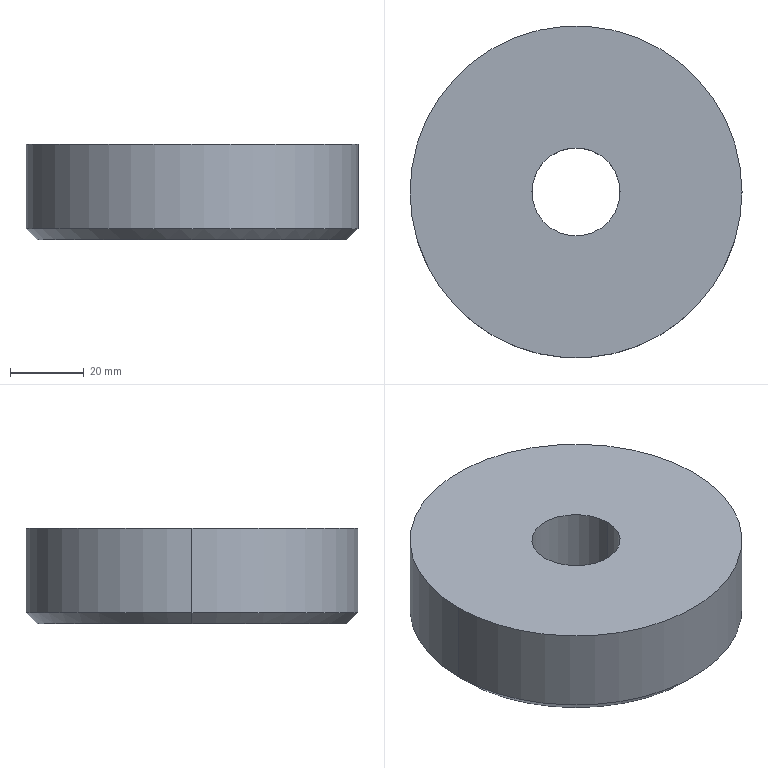Component | SolidWorks | PolishingHead-1 | 1 solid | 8 faces | box 90.34 x 90.34 x 26 mm | volume 153646 mm3 | cylinder 4 | cone 2 | plane 2 | commonest cylinder face diameters 24 x2 90.34 x2
build123d program:
from build123d import *

# Parameters (mm, degrees)
SKETCH1_R           = 45.17
BOSS_EXTRUDE1_DEPTH = 26
CHAMFER1_SIZE       = 3
SKETCH2_R           = 12
CUT_EXTRUDE1_DEPTH  = 26


with BuildPart() as part:
    # Sketch1 → Boss-Extrude1 (new body)
    with BuildSketch(Plane.XY):
        Circle(SKETCH1_R)
    extrude(amount=BOSS_EXTRUDE1_DEPTH)

    # Chamfer1
    chamfer1_edges = [part.edges().sort_by_distance(p)[0] for p in [
        (-45.17, 0, 26),
    ]]
    chamfer(chamfer1_edges, length=CHAMFER1_SIZE)

    # Sketch2 → Cut-Extrude1 (cut)
    with BuildSketch(Plane.XY.offset(26)):
        Circle(SKETCH2_R)
    extrude(amount=-CUT_EXTRUDE1_DEPTH, mode=Mode.SUBTRACT)


solid = part.part

# Placed as in the assembly
solid = solid.moved(Location((0, 0, -90), (180, 0, 0)))
STEP:
#1=CARTESIAN_POINT('',(0.4724,0.,-3.543));
#2=VERTEX_POINT('',#1);
#3=CARTESIAN_POINT('',(-0.4724,0.,-3.543));
#4=VERTEX_POINT('',#3);
#5=CARTESIAN_POINT('',(0.,0.,-3.543));
#6=DIRECTION('',(0.,0.,-1.));
#7=DIRECTION('',(-1.,0.,0.));
#8=AXIS2_PLACEMENT_3D('',#5,#6,#7);
#9=CIRCLE('',#8,0.4724);
#10=EDGE_CURVE('',#2,#4,#9,.T.);
#11=ORIENTED_EDGE('',*,*,#10,.F.);
#12=CARTESIAN_POINT('',(0.4724,0.,-4.567));
#13=VERTEX_POINT('',#12);
#14=CARTESIAN_POINT('',(0.4724,0.,-3.543));
#15=DIRECTION('',(0.,0.,-1.));
#16=VECTOR('',#15,39.37);
#17=LINE('',#14,#16);
#18=EDGE_CURVE('',#2,#13,#17,.T.);
#19=ORIENTED_EDGE('',*,*,#18,.T.);
#20=CARTESIAN_POINT('',(-0.4724,0.,-4.567));
#21=VERTEX_POINT('',#20);
#22=CARTESIAN_POINT('',(0.,0.,-4.567));
#23=DIRECTION('',(0.,0.,-1.));
#24=DIRECTION('',(-1.,0.,0.));
#25=AXIS2_PLACEMENT_3D('',#22,#23,#24);
#26=CIRCLE('',#25,0.4724);
#27=EDGE_CURVE('',#13,#21,#26,.T.);
#28=ORIENTED_EDGE('',*,*,#27,.T.);
#29=CARTESIAN_POINT('',(-0.4724,0.,-3.543));
#30=DIRECTION('',(0.,0.,-1.));
#31=VECTOR('',#30,39.37);
#32=LINE('',#29,#31);
#33=EDGE_CURVE('',#4,#21,#32,.T.);
#34=ORIENTED_EDGE('',*,*,#33,.F.);
#35=EDGE_LOOP('',(#11,#19,#28,#34));
#36=FACE_OUTER_BOUND('',#35,.T.);
#37=CARTESIAN_POINT('',(0.,0.,-3.543));
#38=DIRECTION('',(0.,0.,-1.));
#39=DIRECTION('',(-1.,0.,0.));
#40=AXIS2_PLACEMENT_3D('',#37,#38,#39);
#41=CYLINDRICAL_SURFACE('',#40,0.4724);
#42=ADVANCED_FACE('',(#36),#41,.F.);
#43=CARTESIAN_POINT('',(-1.66,0.,-4.567));
#44=VERTEX_POINT('',#43);
#45=CARTESIAN_POINT('',(1.66,0.,-4.567));
#46=VERTEX_POINT('',#45);
#47=CARTESIAN_POINT('',(0.,0.,-4.567));
#48=DIRECTION('',(0.,0.,-1.));
#49=DIRECTION('',(-1.,0.,0.));
#50=AXIS2_PLACEMENT_3D('',#47,#48,#49);
#51=CIRCLE('',#50,1.66);
#52=EDGE_CURVE('',#44,#46,#51,.T.);
#53=ORIENTED_EDGE('',*,*,#52,.F.);
#54=CARTESIAN_POINT('',(-1.778,0.,-4.449));
#55=VERTEX_POINT('',#54);
#56=CARTESIAN_POINT('',(-1.66,0.,-4.567));
#57=DIRECTION('',(-0.7071,0.,0.7071));
#58=VECTOR('',#57,39.37);
#59=LINE('',#56,#58);
#60=EDGE_CURVE('',#44,#55,#59,.T.);
#61=ORIENTED_EDGE('',*,*,#60,.T.);
#62=CARTESIAN_POINT('',(1.778,0.,-4.449));
#63=VERTEX_POINT('',#62);
#64=CARTESIAN_POINT('',(0.,0.,-4.449));
#65=DIRECTION('',(0.,0.,1.));
#66=DIRECTION('',(-1.,0.,0.));
#67=AXIS2_PLACEMENT_3D('',#64,#65,#66);
#68=CIRCLE('',#67,1.778);
#69=EDGE_CURVE('',#63,#55,#68,.T.);
#70=ORIENTED_EDGE('',*,*,#69,.F.);
#71=CARTESIAN_POINT('',(1.66,0.,-4.567));
#72=DIRECTION('',(0.7071,0.,0.7071));
#73=VECTOR('',#72,39.37);
#74=LINE('',#71,#73);
#75=EDGE_CURVE('',#46,#63,#74,.T.);
#76=ORIENTED_EDGE('',*,*,#75,.F.);
#77=EDGE_LOOP('',(#53,#61,#70,#76));
#78=FACE_OUTER_BOUND('',#77,.T.);
#79=CARTESIAN_POINT('',(0.,0.,-4.567));
#80=DIRECTION('',(0.,0.,1.));
#81=DIRECTION('',(1.,0.,0.));
#82=AXIS2_PLACEMENT_3D('',#79,#80,#81);
#83=CONICAL_SURFACE('',#82,1.66,0.7854);
#84=ADVANCED_FACE('',(#78),#83,.T.);
#85=ORIENTED_EDGE('',*,*,#69,.T.);
#86=CARTESIAN_POINT('',(-1.778,0.,-3.543));
#87=VERTEX_POINT('',#86);
#88=CARTESIAN_POINT('',(-1.778,0.,-4.567));
#89=DIRECTION('',(0.,0.,1.));
#90=VECTOR('',#89,39.37);
#91=LINE('',#88,#90);
#92=EDGE_CURVE('',#55,#87,#91,.T.);
#93=ORIENTED_EDGE('',*,*,#92,.T.);
#94=CARTESIAN_POINT('',(1.778,0.,-3.543));
#95=VERTEX_POINT('',#94);
#96=CARTESIAN_POINT('',(0.,0.,-3.543));
#97=DIRECTION('',(0.,0.,-1.));
#98=DIRECTION('',(-1.,0.,0.));
#99=AXIS2_PLACEMENT_3D('',#96,#97,#98);
#100=CIRCLE('',#99,1.778);
#101=EDGE_CURVE('',#87,#95,#100,.T.);
#102=ORIENTED_EDGE('',*,*,#101,.T.);
#103=CARTESIAN_POINT('',(1.778,0.,-4.567));
#104=DIRECTION('',(0.,0.,1.));
#105=VECTOR('',#104,39.37);
#106=LINE('',#103,#105);
#107=EDGE_CURVE('',#63,#95,#106,.T.);
#108=ORIENTED_EDGE('',*,*,#107,.F.);
#109=EDGE_LOOP('',(#85,#93,#102,#108));
#110=FACE_OUTER_BOUND('',#109,.T.);
#111=CARTESIAN_POINT('',(0.,0.,-4.567));
#112=DIRECTION('',(0.,0.,1.));
#113=DIRECTION('',(1.,0.,0.));
#114=AXIS2_PLACEMENT_3D('',#111,#112,#113);
#115=CYLINDRICAL_SURFACE('',#114,1.778);
#116=ADVANCED_FACE('',(#110),#115,.T.);
#117=ORIENTED_EDGE('',*,*,#92,.F.);
#118=CARTESIAN_POINT('',(0.,0.,-4.449));
#119=DIRECTION('',(0.,0.,1.));
#120=DIRECTION('',(-1.,0.,0.));
#121=AXIS2_PLACEMENT_3D('',#118,#119,#120);
#122=CIRCLE('',#121,1.778);
#123=EDGE_CURVE('',#55,#63,#122,.T.);
#124=ORIENTED_EDGE('',*,*,#123,.T.);
#125=ORIENTED_EDGE('',*,*,#107,.T.);
#126=CARTESIAN_POINT('',(0.,0.,-3.543));
#127=DIRECTION('',(0.,0.,-1.));
#128=DIRECTION('',(-1.,0.,0.));
#129=AXIS2_PLACEMENT_3D('',#126,#127,#128);
#130=CIRCLE('',#129,1.778);
#131=EDGE_CURVE('',#95,#87,#130,.T.);
#132=ORIENTED_EDGE('',*,*,#131,.T.);
#133=EDGE_LOOP('',(#117,#124,#125,#132));
#134=FACE_OUTER_BOUND('',#133,.T.);
#135=CARTESIAN_POINT('',(0.,0.,-4.567));
#136=DIRECTION('',(0.,0.,1.));
#137=DIRECTION('',(1.,0.,0.));
#138=AXIS2_PLACEMENT_3D('',#135,#136,#137);
#139=CYLINDRICAL_SURFACE('',#138,1.778);
#140=ADVANCED_FACE('',(#134),#139,.T.);
#141=CARTESIAN_POINT('',(0.,0.,-4.567));
#142=DIRECTION('',(0.,0.,-1.));
#143=DIRECTION('',(-1.,0.,0.));
#144=AXIS2_PLACEMENT_3D('',#141,#142,#143);
#145=CIRCLE('',#144,0.4724);
#146=EDGE_CURVE('',#21,#13,#145,.T.);
#147=ORIENTED_EDGE('',*,*,#146,.F.);
#148=ORIENTED_EDGE('',*,*,#27,.F.);
#149=EDGE_LOOP('',(#147,#148));
#150=FACE_BOUND('',#149,.T.);
#151=CARTESIAN_POINT('',(0.,0.,-4.567));
#152=DIRECTION('',(0.,0.,-1.));
#153=DIRECTION('',(-1.,0.,0.));
#154=AXIS2_PLACEMENT_3D('',#151,#152,#153);
#155=CIRCLE('',#154,1.66);
#156=EDGE_CURVE('',#46,#44,#155,.T.);
#157=ORIENTED_EDGE('',*,*,#156,.T.);
#158=ORIENTED_EDGE('',*,*,#52,.T.);
#159=EDGE_LOOP('',(#157,#158));
#160=FACE_OUTER_BOUND('',#159,.T.);
#161=CARTESIAN_POINT('',(0.,0.,-4.567));
#162=DIRECTION('',(0.,0.,-1.));
#163=DIRECTION('',(-1.,0.,0.));
#164=AXIS2_PLACEMENT_3D('',#161,#162,#163);
#165=PLANE('',#164);
#166=ADVANCED_FACE('',(#150,#160),#165,.T.);
#167=CARTESIAN_POINT('',(0.,0.,-3.543));
#168=DIRECTION('',(0.,0.,-1.));
#169=DIRECTION('',(-1.,0.,0.));
#170=AXIS2_PLACEMENT_3D('',#167,#168,#169);
#171=CIRCLE('',#170,0.4724);
#172=EDGE_CURVE('',#4,#2,#171,.T.);
#173=ORIENTED_EDGE('',*,*,#172,.T.);
#174=ORIENTED_EDGE('',*,*,#10,.T.);
#175=EDGE_LOOP('',(#173,#174));
#176=FACE_BOUND('',#175,.T.);
#177=ORIENTED_EDGE('',*,*,#131,.F.);
#178=ORIENTED_EDGE('',*,*,#101,.F.);
#179=EDGE_LOOP('',(#177,#178));
#180=FACE_OUTER_BOUND('',#179,.T.);
#181=CARTESIAN_POINT('',(0.,0.,-3.543));
#182=DIRECTION('',(0.,0.,-1.));
#183=DIRECTION('',(-1.,0.,0.));
#184=AXIS2_PLACEMENT_3D('',#181,#182,#183);
#185=PLANE('',#184);
#186=ADVANCED_FACE('',(#176,#180),#185,.F.);
#187=ORIENTED_EDGE('',*,*,#60,.F.);
#188=ORIENTED_EDGE('',*,*,#156,.F.);
#189=ORIENTED_EDGE('',*,*,#75,.T.);
#190=ORIENTED_EDGE('',*,*,#123,.F.);
#191=EDGE_LOOP('',(#187,#188,#189,#190));
#192=FACE_OUTER_BOUND('',#191,.T.);
#193=CARTESIAN_POINT('',(0.,0.,-4.567));
#194=DIRECTION('',(0.,0.,1.));
#195=DIRECTION('',(1.,0.,0.));
#196=AXIS2_PLACEMENT_3D('',#193,#194,#195);
#197=CONICAL_SURFACE('',#196,1.66,0.7854);
#198=ADVANCED_FACE('',(#192),#197,.T.);
#199=ORIENTED_EDGE('',*,*,#18,.F.);
#200=ORIENTED_EDGE('',*,*,#172,.F.);
#201=ORIENTED_EDGE('',*,*,#33,.T.);
#202=ORIENTED_EDGE('',*,*,#146,.T.);
#203=EDGE_LOOP('',(#199,#200,#201,#202));
#204=FACE_OUTER_BOUND('',#203,.T.);
#205=CARTESIAN_POINT('',(0.,0.,-3.543));
#206=DIRECTION('',(0.,0.,-1.));
#207=DIRECTION('',(-1.,0.,0.));
#208=AXIS2_PLACEMENT_3D('',#205,#206,#207);
#209=CYLINDRICAL_SURFACE('',#208,0.4724);
#210=ADVANCED_FACE('',(#204),#209,.F.);
#211=CLOSED_SHELL('',(#42,#84,#116,#140,#166,#186,#198,#210));
#212=MANIFOLD_SOLID_BREP('',#211);
#213=CARTESIAN_POINT('',(0.,0.,0.));
#214=DIRECTION('',(0.,0.,1.));
#215=DIRECTION('',(1.,0.,0.));
#216=AXIS2_PLACEMENT_3D('',#213,#214,#215);
#217=(LENGTH_UNIT()NAMED_UNIT(*)SI_UNIT($,.METRE.));
#218=LENGTH_MEASURE_WITH_UNIT(LENGTH_MEASURE(0.0254),#217);
#219=DIMENSIONAL_EXPONENTS(1.,0.,0.,0.,0.,0.,0.);
#220=(CONVERSION_BASED_UNIT('',#218)LENGTH_UNIT()NAMED_UNIT(#219));
#221=UNCERTAINTY_MEASURE_WITH_UNIT(LENGTH_MEASURE(0.00001),#220,'','');
#222=(NAMED_UNIT(*)PLANE_ANGLE_UNIT()SI_UNIT($,.RADIAN.));
#223=(NAMED_UNIT(*)SI_UNIT($,.STERADIAN.)SOLID_ANGLE_UNIT());
#224=(GEOMETRIC_REPRESENTATION_CONTEXT(3)GLOBAL_UNCERTAINTY_ASSIGNED_CONTEXT((#221))GLOBAL_UNIT_ASSIGNED_CONTEXT((#220,#222,#223))REPRESENTATION_CONTEXT('',''));
#225=ADVANCED_BREP_SHAPE_REPRESENTATION('',(#212,#216),#224);
#226=COLOUR_RGB('',0.7922,0.8196,0.9333);
#227=FILL_AREA_STYLE_COLOUR('',#226);
#228=FILL_AREA_STYLE('',(#227));
#229=SURFACE_STYLE_FILL_AREA(#228);
#230=SURFACE_SIDE_STYLE('',(#229));
#231=SURFACE_STYLE_USAGE(.BOTH.,#230);
#232=PRESENTATION_STYLE_ASSIGNMENT((#231));
#233=STYLED_ITEM('',(#232),#212);
#234=(LENGTH_UNIT()NAMED_UNIT(*)SI_UNIT($,.METRE.));
#235=LENGTH_MEASURE_WITH_UNIT(LENGTH_MEASURE(0.0254),#234);
#236=DIMENSIONAL_EXPONENTS(1.,0.,0.,0.,0.,0.,0.);
#237=(CONVERSION_BASED_UNIT('',#235)LENGTH_UNIT()NAMED_UNIT(#236));
#238=UNCERTAINTY_MEASURE_WITH_UNIT(LENGTH_MEASURE(0.00001),#237,'','');
#239=(NAMED_UNIT(*)PLANE_ANGLE_UNIT()SI_UNIT($,.RADIAN.));
#240=(NAMED_UNIT(*)SI_UNIT($,.STERADIAN.)SOLID_ANGLE_UNIT());
#241=(GEOMETRIC_REPRESENTATION_CONTEXT(3)GLOBAL_UNCERTAINTY_ASSIGNED_CONTEXT((#238))GLOBAL_UNIT_ASSIGNED_CONTEXT((#237,#239,#240))REPRESENTATION_CONTEXT('',''));
#242=MECHANICAL_DESIGN_GEOMETRIC_PRESENTATION_REPRESENTATION('',(#233),#241);
#243=PRESENTATION_LAYER_ASSIGNMENT('','',(#233));